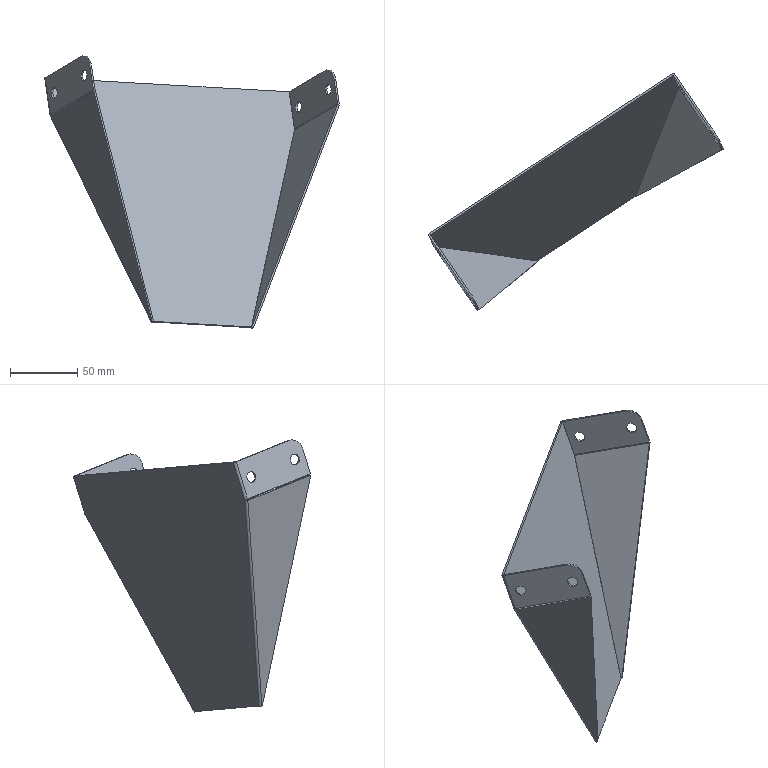Component | SolidWorks | MaterialGate-1 | 1 solid | 50 faces | volume 67130 mm3 | plane 26 | cylinder 18 | spline 6 | commonest cylinder face diameters 8 x8 0.2 x4 3.2 x4 20 x2 | material AISI 304